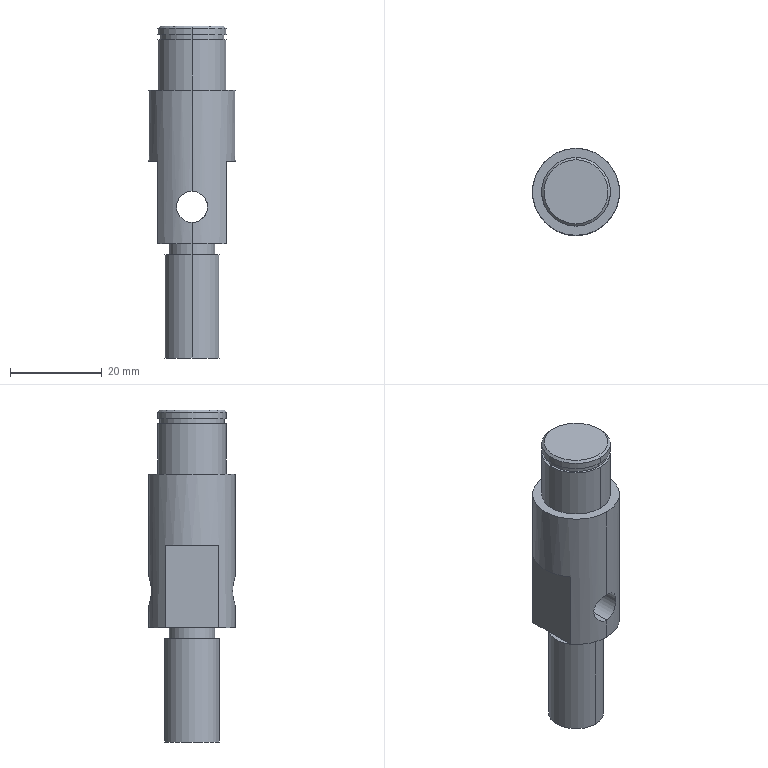Component | SolidWorks | DoubleFilmTransport-1_TensionConnectionAxis-1 | 1 solid | 27 faces | box 19 x 19 x 72.5 mm | volume 13431 mm3 | cylinder 14 | plane 11 | cone 2 | commonest cylinder face diameters 15 x4 6.8 x2 12 x2 10 x2 19 x2 14 x2
STEP:
#1=CARTESIAN_POINT('',(-15.145,10.074,3.252));
#2=VERTEX_POINT('',#1);
#3=CARTESIAN_POINT('',(-15.145,10.074,3.52));
#4=VERTEX_POINT('',#3);
#5=CARTESIAN_POINT('',(-15.145,10.074,3.252));
#6=CARTESIAN_POINT('',(-15.136,10.074,3.252));
#7=CARTESIAN_POINT('',(-15.127,10.074,3.253));
#8=CARTESIAN_POINT('',(-15.11,10.075,3.256));
#9=CARTESIAN_POINT('',(-15.101,10.076,3.259));
#10=CARTESIAN_POINT('',(-15.085,10.078,3.266));
#11=CARTESIAN_POINT('',(-15.077,10.08,3.27));
#12=CARTESIAN_POINT('',(-15.063,10.083,3.279));
#13=CARTESIAN_POINT('',(-15.056,10.084,3.285));
#14=CARTESIAN_POINT('',(-15.038,10.089,3.303));
#15=CARTESIAN_POINT('',(-15.028,10.092,3.318));
#16=CARTESIAN_POINT('',(-15.018,10.096,3.342));
#17=CARTESIAN_POINT('',(-15.015,10.097,3.351));
#18=CARTESIAN_POINT('',(-15.012,10.098,3.368));
#19=CARTESIAN_POINT('',(-15.011,10.099,3.377));
#20=CARTESIAN_POINT('',(-15.011,10.099,3.395));
#21=CARTESIAN_POINT('',(-15.012,10.098,3.404));
#22=CARTESIAN_POINT('',(-15.015,10.097,3.421));
#23=CARTESIAN_POINT('',(-15.018,10.096,3.429));
#24=CARTESIAN_POINT('',(-15.025,10.094,3.445));
#25=CARTESIAN_POINT('',(-15.029,10.092,3.453));
#26=CARTESIAN_POINT('',(-15.038,10.089,3.468));
#27=CARTESIAN_POINT('',(-15.044,10.088,3.474));
#28=CARTESIAN_POINT('',(-15.056,10.084,3.487));
#29=CARTESIAN_POINT('',(-15.063,10.083,3.492));
#30=CARTESIAN_POINT('',(-15.077,10.08,3.502));
#31=CARTESIAN_POINT('',(-15.085,10.078,3.506));
#32=CARTESIAN_POINT('',(-15.101,10.076,3.513));
#33=CARTESIAN_POINT('',(-15.11,10.075,3.515));
#34=CARTESIAN_POINT('',(-15.127,10.074,3.519));
#35=CARTESIAN_POINT('',(-15.136,10.074,3.52));
#36=CARTESIAN_POINT('',(-15.145,10.074,3.52));
#37=B_SPLINE_CURVE_WITH_KNOTS('',3,(#5,#6,#7,#8,#9,#10,#11,#12,#13,#14,#15,#16,#17,#18,#19,#20,#21,#22,#23,#24,#25,#26,#27,#28,#29,#30,#31,#32,#33,#34,#35,#36),.UNSPECIFIED.,.F.,.F.,(4,2,2,2,2,2,2,2,2,2,2,2,2,2,2,4),(0.,0.00067,0.00134,0.00201,0.00268,0.00402,0.00469,0.00536,0.00603,0.0067,0.00737,0.00804,0.00871,0.00938,0.01005,0.01072),.UNSPECIFIED.);
#38=EDGE_CURVE('',#2,#4,#37,.T.);
#39=ORIENTED_EDGE('',*,*,#38,.T.);
#40=CARTESIAN_POINT('',(-15.145,10.822,3.52));
#41=VERTEX_POINT('',#40);
#42=CARTESIAN_POINT('',(-15.145,10.822,3.52));
#43=DIRECTION('',(0.,1.,0.));
#44=VECTOR('',#43,39.37);
#45=LINE('',#42,#44);
#46=EDGE_CURVE('',#4,#41,#45,.T.);
#47=ORIENTED_EDGE('',*,*,#46,.T.);
#48=CARTESIAN_POINT('',(-15.145,10.822,3.252));
#49=VERTEX_POINT('',#48);
#50=CARTESIAN_POINT('',(-15.145,10.822,3.52));
#51=CARTESIAN_POINT('',(-15.136,10.822,3.52));
#52=CARTESIAN_POINT('',(-15.127,10.821,3.519));
#53=CARTESIAN_POINT('',(-15.11,10.82,3.515));
#54=CARTESIAN_POINT('',(-15.101,10.819,3.513));
#55=CARTESIAN_POINT('',(-15.085,10.817,3.506));
#56=CARTESIAN_POINT('',(-15.077,10.816,3.502));
#57=CARTESIAN_POINT('',(-15.063,10.813,3.492));
#58=CARTESIAN_POINT('',(-15.056,10.811,3.487));
#59=CARTESIAN_POINT('',(-15.044,10.808,3.474));
#60=CARTESIAN_POINT('',(-15.038,10.806,3.468));
#61=CARTESIAN_POINT('',(-15.029,10.803,3.453));
#62=CARTESIAN_POINT('',(-15.025,10.802,3.445));
#63=CARTESIAN_POINT('',(-15.018,10.8,3.429));
#64=CARTESIAN_POINT('',(-15.015,10.799,3.421));
#65=CARTESIAN_POINT('',(-15.012,10.797,3.404));
#66=CARTESIAN_POINT('',(-15.011,10.797,3.395));
#67=CARTESIAN_POINT('',(-15.011,10.797,3.377));
#68=CARTESIAN_POINT('',(-15.012,10.797,3.368));
#69=CARTESIAN_POINT('',(-15.015,10.799,3.351));
#70=CARTESIAN_POINT('',(-15.018,10.8,3.342));
#71=CARTESIAN_POINT('',(-15.025,10.802,3.326));
#72=CARTESIAN_POINT('',(-15.029,10.803,3.319));
#73=CARTESIAN_POINT('',(-15.038,10.806,3.304));
#74=CARTESIAN_POINT('',(-15.044,10.808,3.297));
#75=CARTESIAN_POINT('',(-15.056,10.811,3.285));
#76=CARTESIAN_POINT('',(-15.063,10.813,3.279));
#77=CARTESIAN_POINT('',(-15.078,10.816,3.27));
#78=CARTESIAN_POINT('',(-15.085,10.817,3.266));
#79=CARTESIAN_POINT('',(-15.101,10.819,3.259));
#80=CARTESIAN_POINT('',(-15.11,10.82,3.256));
#81=CARTESIAN_POINT('',(-15.127,10.821,3.253));
#82=CARTESIAN_POINT('',(-15.136,10.822,3.252));
#83=CARTESIAN_POINT('',(-15.145,10.822,3.252));
#84=B_SPLINE_CURVE_WITH_KNOTS('',3,(#50,#51,#52,#53,#54,#55,#56,#57,#58,#59,#60,#61,#62,#63,#64,#65,#66,#67,#68,#69,#70,#71,#72,#73,#74,#75,#76,#77,#78,#79,#80,#81,#82,#83),.UNSPECIFIED.,.F.,.F.,(4,2,2,2,2,2,2,2,2,2,2,2,2,2,2,2,4),(0.01072,0.01139,0.01206,0.01273,0.0134,0.01407,0.01474,0.01541,0.01608,0.01675,0.01742,0.01809,0.01876,0.01943,0.0201,0.02077,0.02144),.UNSPECIFIED.);
#85=EDGE_CURVE('',#41,#49,#84,.T.);
#86=ORIENTED_EDGE('',*,*,#85,.T.);
#87=CARTESIAN_POINT('',(-15.145,10.822,3.252));
#88=DIRECTION('',(0.,1.,0.));
#89=VECTOR('',#88,39.37);
#90=LINE('',#87,#89);
#91=EDGE_CURVE('',#2,#49,#90,.T.);
#92=ORIENTED_EDGE('',*,*,#91,.F.);
#93=EDGE_LOOP('',(#39,#47,#86,#92));
#94=FACE_OUTER_BOUND('',#93,.T.);
#95=CARTESIAN_POINT('',(-15.145,10.822,3.386));
#96=DIRECTION('',(0.,1.,0.));
#97=DIRECTION('',(0.,0.,-1.));
#98=AXIS2_PLACEMENT_3D('',#95,#96,#97);
#99=CYLINDRICAL_SURFACE('',#98,0.1339);
#100=ADVANCED_FACE('',(#94),#99,.F.);
#101=CARTESIAN_POINT('',(-15.145,10.684,2.087));
#102=VERTEX_POINT('',#101);
#103=CARTESIAN_POINT('',(-15.145,10.212,2.087));
#104=VERTEX_POINT('',#103);
#105=CARTESIAN_POINT('',(-15.145,10.448,2.087));
#106=DIRECTION('',(0.,0.,1.));
#107=DIRECTION('',(0.,-1.,0.));
#108=AXIS2_PLACEMENT_3D('',#105,#106,#107);
#109=CIRCLE('',#108,0.2362);
#110=EDGE_CURVE('',#102,#104,#109,.T.);
#111=ORIENTED_EDGE('',*,*,#110,.T.);
#112=CARTESIAN_POINT('',(-15.145,10.212,2.972));
#113=VERTEX_POINT('',#112);
#114=CARTESIAN_POINT('',(-15.145,10.212,2.087));
#115=DIRECTION('',(0.,0.,1.));
#116=VECTOR('',#115,39.37);
#117=LINE('',#114,#116);
#118=EDGE_CURVE('',#104,#113,#117,.T.);
#119=ORIENTED_EDGE('',*,*,#118,.T.);
#120=CARTESIAN_POINT('',(-15.145,10.684,2.972));
#121=VERTEX_POINT('',#120);
#122=CARTESIAN_POINT('',(-15.145,10.448,2.972));
#123=DIRECTION('',(0.,0.,1.));
#124=DIRECTION('',(0.,-1.,0.));
#125=AXIS2_PLACEMENT_3D('',#122,#123,#124);
#126=CIRCLE('',#125,0.2362);
#127=EDGE_CURVE('',#121,#113,#126,.T.);
#128=ORIENTED_EDGE('',*,*,#127,.F.);
#129=CARTESIAN_POINT('',(-15.145,10.684,2.087));
#130=DIRECTION('',(0.,0.,1.));
#131=VECTOR('',#130,39.37);
#132=LINE('',#129,#131);
#133=EDGE_CURVE('',#102,#121,#132,.T.);
#134=ORIENTED_EDGE('',*,*,#133,.F.);
#135=EDGE_LOOP('',(#111,#119,#128,#134));
#136=FACE_OUTER_BOUND('',#135,.T.);
#137=CARTESIAN_POINT('',(-15.145,10.448,2.087));
#138=DIRECTION('',(0.,0.,1.));
#139=DIRECTION('',(0.,1.,0.));
#140=AXIS2_PLACEMENT_3D('',#137,#138,#139);
#141=CYLINDRICAL_SURFACE('',#140,0.2362);
#142=ADVANCED_FACE('',(#136),#141,.T.);
#143=CARTESIAN_POINT('',(-15.145,10.251,2.972));
#144=VERTEX_POINT('',#143);
#145=CARTESIAN_POINT('',(-15.145,10.645,2.972));
#146=VERTEX_POINT('',#145);
#147=CARTESIAN_POINT('',(-15.145,10.448,2.972));
#148=DIRECTION('',(0.,0.,-1.));
#149=DIRECTION('',(0.,-1.,0.));
#150=AXIS2_PLACEMENT_3D('',#147,#148,#149);
#151=CIRCLE('',#150,0.1969);
#152=EDGE_CURVE('',#144,#146,#151,.T.);
#153=ORIENTED_EDGE('',*,*,#152,.F.);
#154=CARTESIAN_POINT('',(-15.145,10.251,3.071));
#155=VERTEX_POINT('',#154);
#156=CARTESIAN_POINT('',(-15.145,10.251,2.972));
#157=DIRECTION('',(0.,0.,1.));
#158=VECTOR('',#157,39.37);
#159=LINE('',#156,#158);
#160=EDGE_CURVE('',#144,#155,#159,.T.);
#161=ORIENTED_EDGE('',*,*,#160,.T.);
#162=CARTESIAN_POINT('',(-15.145,10.645,3.071));
#163=VERTEX_POINT('',#162);
#164=CARTESIAN_POINT('',(-15.145,10.448,3.071));
#165=DIRECTION('',(0.,0.,-1.));
#166=DIRECTION('',(0.,-1.,0.));
#167=AXIS2_PLACEMENT_3D('',#164,#165,#166);
#168=CIRCLE('',#167,0.1969);
#169=EDGE_CURVE('',#155,#163,#168,.T.);
#170=ORIENTED_EDGE('',*,*,#169,.T.);
#171=CARTESIAN_POINT('',(-15.145,10.645,2.972));
#172=DIRECTION('',(0.,0.,1.));
#173=VECTOR('',#172,39.37);
#174=LINE('',#171,#173);
#175=EDGE_CURVE('',#146,#163,#174,.T.);
#176=ORIENTED_EDGE('',*,*,#175,.F.);
#177=EDGE_LOOP('',(#153,#161,#170,#176));
#178=FACE_OUTER_BOUND('',#177,.T.);
#179=CARTESIAN_POINT('',(-15.145,10.448,2.972));
#180=DIRECTION('',(0.,0.,1.));
#181=DIRECTION('',(0.,1.,0.));
#182=AXIS2_PLACEMENT_3D('',#179,#180,#181);
#183=CYLINDRICAL_SURFACE('',#182,0.1969);
#184=ADVANCED_FACE('',(#178),#183,.T.);
#185=CARTESIAN_POINT('',(-15.44,10.218,3.071));
#186=VERTEX_POINT('',#185);
#187=CARTESIAN_POINT('',(-15.145,10.074,3.071));
#188=VERTEX_POINT('',#187);
#189=CARTESIAN_POINT('',(-15.145,10.448,3.071));
#190=DIRECTION('',(0.,0.,1.));
#191=DIRECTION('',(0.,-1.,0.));
#192=AXIS2_PLACEMENT_3D('',#189,#190,#191);
#193=CIRCLE('',#192,0.374);
#194=EDGE_CURVE('',#186,#188,#193,.T.);
#195=ORIENTED_EDGE('',*,*,#194,.T.);
#196=CARTESIAN_POINT('',(-15.145,10.074,3.071));
#197=DIRECTION('',(0.,0.,1.));
#198=VECTOR('',#197,39.37);
#199=LINE('',#196,#198);
#200=EDGE_CURVE('',#188,#2,#199,.T.);
#201=ORIENTED_EDGE('',*,*,#200,.T.);
#202=CARTESIAN_POINT('',(-15.145,10.074,3.52));
#203=CARTESIAN_POINT('',(-15.154,10.074,3.52));
#204=CARTESIAN_POINT('',(-15.162,10.074,3.519));
#205=CARTESIAN_POINT('',(-15.18,10.075,3.515));
#206=CARTESIAN_POINT('',(-15.188,10.076,3.513));
#207=CARTESIAN_POINT('',(-15.204,10.078,3.506));
#208=CARTESIAN_POINT('',(-15.212,10.08,3.502));
#209=CARTESIAN_POINT('',(-15.227,10.083,3.492));
#210=CARTESIAN_POINT('',(-15.233,10.084,3.487));
#211=CARTESIAN_POINT('',(-15.246,10.088,3.474));
#212=CARTESIAN_POINT('',(-15.251,10.089,3.468));
#213=CARTESIAN_POINT('',(-15.261,10.092,3.453));
#214=CARTESIAN_POINT('',(-15.265,10.094,3.445));
#215=CARTESIAN_POINT('',(-15.272,10.096,3.429));
#216=CARTESIAN_POINT('',(-15.274,10.097,3.421));
#217=CARTESIAN_POINT('',(-15.278,10.098,3.404));
#218=CARTESIAN_POINT('',(-15.279,10.099,3.395));
#219=CARTESIAN_POINT('',(-15.279,10.099,3.377));
#220=CARTESIAN_POINT('',(-15.278,10.098,3.368));
#221=CARTESIAN_POINT('',(-15.274,10.097,3.351));
#222=CARTESIAN_POINT('',(-15.272,10.096,3.342));
#223=CARTESIAN_POINT('',(-15.265,10.094,3.326));
#224=CARTESIAN_POINT('',(-15.261,10.092,3.319));
#225=CARTESIAN_POINT('',(-15.251,10.089,3.304));
#226=CARTESIAN_POINT('',(-15.246,10.088,3.297));
#227=CARTESIAN_POINT('',(-15.233,10.084,3.285));
#228=CARTESIAN_POINT('',(-15.226,10.083,3.279));
#229=CARTESIAN_POINT('',(-15.212,10.08,3.27));
#230=CARTESIAN_POINT('',(-15.204,10.078,3.266));
#231=CARTESIAN_POINT('',(-15.188,10.076,3.259));
#232=CARTESIAN_POINT('',(-15.18,10.075,3.256));
#233=CARTESIAN_POINT('',(-15.162,10.074,3.253));
#234=CARTESIAN_POINT('',(-15.154,10.074,3.252));
#235=CARTESIAN_POINT('',(-15.145,10.074,3.252));
#236=B_SPLINE_CURVE_WITH_KNOTS('',3,(#202,#203,#204,#205,#206,#207,#208,#209,#210,#211,#212,#213,#214,#215,#216,#217,#218,#219,#220,#221,#222,#223,#224,#225,#226,#227,#228,#229,#230,#231,#232,#233,#234,#235),.UNSPECIFIED.,.F.,.F.,(4,2,2,2,2,2,2,2,2,2,2,2,2,2,2,2,4),(0.01072,0.01139,0.01206,0.01273,0.0134,0.01407,0.01474,0.01541,0.01608,0.01675,0.01742,0.01809,0.01876,0.01943,0.0201,0.02077,0.02144),.UNSPECIFIED.);
#237=EDGE_CURVE('',#4,#2,#236,.T.);
#238=ORIENTED_EDGE('',*,*,#237,.F.);
#239=CARTESIAN_POINT('',(-15.145,10.074,4.39));
#240=VERTEX_POINT('',#239);
#241=CARTESIAN_POINT('',(-15.145,10.074,3.071));
#242=DIRECTION('',(0.,0.,1.));
#243=VECTOR('',#242,39.37);
#244=LINE('',#241,#243);
#245=EDGE_CURVE('',#4,#240,#244,.T.);
#246=ORIENTED_EDGE('',*,*,#245,.T.);
#247=CARTESIAN_POINT('',(-15.145,10.822,4.39));
#248=VERTEX_POINT('',#247);
#249=CARTESIAN_POINT('',(-15.145,10.448,4.39));
#250=DIRECTION('',(0.,0.,1.));
#251=DIRECTION('',(0.,-1.,0.));
#252=AXIS2_PLACEMENT_3D('',#249,#250,#251);
#253=CIRCLE('',#252,0.374);
#254=EDGE_CURVE('',#248,#240,#253,.T.);
#255=ORIENTED_EDGE('',*,*,#254,.F.);
#256=CARTESIAN_POINT('',(-15.145,10.822,3.071));
#257=DIRECTION('',(0.,0.,1.));
#258=VECTOR('',#257,39.37);
#259=LINE('',#256,#258);
#260=EDGE_CURVE('',#41,#248,#259,.T.);
#261=ORIENTED_EDGE('',*,*,#260,.F.);
#262=CARTESIAN_POINT('',(-15.145,10.822,3.252));
#263=CARTESIAN_POINT('',(-15.154,10.822,3.252));
#264=CARTESIAN_POINT('',(-15.162,10.821,3.253));
#265=CARTESIAN_POINT('',(-15.18,10.82,3.256));
#266=CARTESIAN_POINT('',(-15.188,10.819,3.259));
#267=CARTESIAN_POINT('',(-15.204,10.817,3.266));
#268=CARTESIAN_POINT('',(-15.212,10.816,3.27));
#269=CARTESIAN_POINT('',(-15.227,10.813,3.279));
#270=CARTESIAN_POINT('',(-15.233,10.811,3.285));
#271=CARTESIAN_POINT('',(-15.252,10.806,3.303));
#272=CARTESIAN_POINT('',(-15.262,10.803,3.318));
#273=CARTESIAN_POINT('',(-15.272,10.8,3.342));
#274=CARTESIAN_POINT('',(-15.274,10.799,3.351));
#275=CARTESIAN_POINT('',(-15.278,10.797,3.368));
#276=CARTESIAN_POINT('',(-15.279,10.797,3.377));
#277=CARTESIAN_POINT('',(-15.279,10.797,3.395));
#278=CARTESIAN_POINT('',(-15.278,10.797,3.404));
#279=CARTESIAN_POINT('',(-15.274,10.799,3.421));
#280=CARTESIAN_POINT('',(-15.272,10.8,3.429));
#281=CARTESIAN_POINT('',(-15.265,10.802,3.445));
#282=CARTESIAN_POINT('',(-15.261,10.803,3.453));
#283=CARTESIAN_POINT('',(-15.251,10.806,3.468));
#284=CARTESIAN_POINT('',(-15.246,10.808,3.474));
#285=CARTESIAN_POINT('',(-15.233,10.811,3.487));
#286=CARTESIAN_POINT('',(-15.227,10.813,3.492));
#287=CARTESIAN_POINT('',(-15.212,10.816,3.502));
#288=CARTESIAN_POINT('',(-15.204,10.817,3.506));
#289=CARTESIAN_POINT('',(-15.188,10.819,3.513));
#290=CARTESIAN_POINT('',(-15.18,10.82,3.515));
#291=CARTESIAN_POINT('',(-15.162,10.821,3.519));
#292=CARTESIAN_POINT('',(-15.154,10.822,3.52));
#293=CARTESIAN_POINT('',(-15.145,10.822,3.52));
#294=B_SPLINE_CURVE_WITH_KNOTS('',3,(#262,#263,#264,#265,#266,#267,#268,#269,#270,#271,#272,#273,#274,#275,#276,#277,#278,#279,#280,#281,#282,#283,#284,#285,#286,#287,#288,#289,#290,#291,#292,#293),.UNSPECIFIED.,.F.,.F.,(4,2,2,2,2,2,2,2,2,2,2,2,2,2,2,4),(0.,0.00067,0.00134,0.00201,0.00268,0.00402,0.00469,0.00536,0.00603,0.0067,0.00737,0.00804,0.00871,0.00938,0.01005,0.01072),.UNSPECIFIED.);
#295=EDGE_CURVE('',#49,#41,#294,.T.);
#296=ORIENTED_EDGE('',*,*,#295,.F.);
#297=CARTESIAN_POINT('',(-15.145,10.822,3.071));
#298=VERTEX_POINT('',#297);
#299=CARTESIAN_POINT('',(-15.145,10.822,3.071));
#300=DIRECTION('',(0.,0.,1.));
#301=VECTOR('',#300,39.37);
#302=LINE('',#299,#301);
#303=EDGE_CURVE('',#298,#49,#302,.T.);
#304=ORIENTED_EDGE('',*,*,#303,.F.);
#305=CARTESIAN_POINT('',(-15.44,10.677,3.071));
#306=VERTEX_POINT('',#305);
#307=CARTESIAN_POINT('',(-15.145,10.448,3.071));
#308=DIRECTION('',(0.,0.,1.));
#309=DIRECTION('',(0.,-1.,0.));
#310=AXIS2_PLACEMENT_3D('',#307,#308,#309);
#311=CIRCLE('',#310,0.374);
#312=EDGE_CURVE('',#298,#306,#311,.T.);
#313=ORIENTED_EDGE('',*,*,#312,.T.);
#314=CARTESIAN_POINT('',(-15.44,10.677,3.78));
#315=VERTEX_POINT('',#314);
#316=CARTESIAN_POINT('',(-15.44,10.677,3.78));
#317=DIRECTION('',(0.,0.,-1.));
#318=VECTOR('',#317,39.37);
#319=LINE('',#316,#318);
#320=EDGE_CURVE('',#315,#306,#319,.T.);
#321=ORIENTED_EDGE('',*,*,#320,.F.);
#322=CARTESIAN_POINT('',(-15.44,10.218,3.78));
#323=VERTEX_POINT('',#322);
#324=CARTESIAN_POINT('',(-15.145,10.448,3.78));
#325=DIRECTION('',(0.,0.,-1.));
#326=DIRECTION('',(0.,-1.,0.));
#327=AXIS2_PLACEMENT_3D('',#324,#325,#326);
#328=CIRCLE('',#327,0.374);
#329=EDGE_CURVE('',#323,#315,#328,.T.);
#330=ORIENTED_EDGE('',*,*,#329,.F.);
#331=CARTESIAN_POINT('',(-15.44,10.218,3.78));
#332=DIRECTION('',(0.,0.,-1.));
#333=VECTOR('',#332,39.37);
#334=LINE('',#331,#333);
#335=EDGE_CURVE('',#323,#186,#334,.T.);
#336=ORIENTED_EDGE('',*,*,#335,.T.);
#337=EDGE_LOOP('',(#195,#201,#238,#246,#255,#261,#296,#304,#313,#321,#330,#336));
#338=FACE_OUTER_BOUND('',#337,.T.);
#339=CARTESIAN_POINT('',(-15.145,10.448,3.071));
#340=DIRECTION('',(0.,0.,1.));
#341=DIRECTION('',(0.,1.,0.));
#342=AXIS2_PLACEMENT_3D('',#339,#340,#341);
#343=CYLINDRICAL_SURFACE('',#342,0.374);
#344=ADVANCED_FACE('',(#338),#343,.T.);
#345=CARTESIAN_POINT('',(-15.145,10.743,4.39));
#346=VERTEX_POINT('',#345);
#347=CARTESIAN_POINT('',(-15.145,10.152,4.39));
#348=VERTEX_POINT('',#347);
#349=CARTESIAN_POINT('',(-15.145,10.448,4.39));
#350=DIRECTION('',(0.,0.,1.));
#351=DIRECTION('',(0.,-1.,0.));
#352=AXIS2_PLACEMENT_3D('',#349,#350,#351);
#353=CIRCLE('',#352,0.2953);
#354=EDGE_CURVE('',#346,#348,#353,.T.);
#355=ORIENTED_EDGE('',*,*,#354,.T.);
#356=CARTESIAN_POINT('',(-15.145,10.152,4.823));
#357=VERTEX_POINT('',#356);
#358=CARTESIAN_POINT('',(-15.145,10.152,4.39));
#359=DIRECTION('',(0.,0.,1.));
#360=VECTOR('',#359,39.37);
#361=LINE('',#358,#360);
#362=EDGE_CURVE('',#348,#357,#361,.T.);
#363=ORIENTED_EDGE('',*,*,#362,.T.);
#364=CARTESIAN_POINT('',(-15.145,10.743,4.823));
#365=VERTEX_POINT('',#364);
#366=CARTESIAN_POINT('',(-15.145,10.448,4.823));
#367=DIRECTION('',(0.,0.,1.));
#368=DIRECTION('',(0.,-1.,0.));
#369=AXIS2_PLACEMENT_3D('',#366,#367,#368);
#370=CIRCLE('',#369,0.2953);
#371=EDGE_CURVE('',#365,#357,#370,.T.);
#372=ORIENTED_EDGE('',*,*,#371,.F.);
#373=CARTESIAN_POINT('',(-15.145,10.743,4.39));
#374=DIRECTION('',(0.,0.,1.));
#375=VECTOR('',#374,39.37);
#376=LINE('',#373,#375);
#377=EDGE_CURVE('',#346,#365,#376,.T.);
#378=ORIENTED_EDGE('',*,*,#377,.F.);
#379=EDGE_LOOP('',(#355,#363,#372,#378));
#380=FACE_OUTER_BOUND('',#379,.T.);
#381=CARTESIAN_POINT('',(-15.145,10.448,4.39));
#382=DIRECTION('',(0.,0.,1.));
#383=DIRECTION('',(0.,1.,0.));
#384=AXIS2_PLACEMENT_3D('',#381,#382,#383);
#385=CYLINDRICAL_SURFACE('',#384,0.2953);
#386=ADVANCED_FACE('',(#380),#385,.T.);
#387=CARTESIAN_POINT('',(-15.145,10.172,4.823));
#388=VERTEX_POINT('',#387);
#389=CARTESIAN_POINT('',(-15.145,10.723,4.823));
#390=VERTEX_POINT('',#389);
#391=CARTESIAN_POINT('',(-15.145,10.448,4.823));
#392=DIRECTION('',(0.,0.,-1.));
#393=DIRECTION('',(0.,-1.,0.));
#394=AXIS2_PLACEMENT_3D('',#391,#392,#393);
#395=CIRCLE('',#394,0.2756);
#396=EDGE_CURVE('',#388,#390,#395,.T.);
#397=ORIENTED_EDGE('',*,*,#396,.F.);
#398=CARTESIAN_POINT('',(-15.145,10.172,4.866));
#399=VERTEX_POINT('',#398);
#400=CARTESIAN_POINT('',(-15.145,10.172,4.823));
#401=DIRECTION('',(0.,0.,1.));
#402=VECTOR('',#401,39.37);
#403=LINE('',#400,#402);
#404=EDGE_CURVE('',#388,#399,#403,.T.);
#405=ORIENTED_EDGE('',*,*,#404,.T.);
#406=CARTESIAN_POINT('',(-15.145,10.723,4.866));
#407=VERTEX_POINT('',#406);
#408=CARTESIAN_POINT('',(-15.145,10.448,4.866));
#409=DIRECTION('',(0.,0.,-1.));
#410=DIRECTION('',(0.,-1.,0.));
#411=AXIS2_PLACEMENT_3D('',#408,#409,#410);
#412=CIRCLE('',#411,0.2756);
#413=EDGE_CURVE('',#399,#407,#412,.T.);
#414=ORIENTED_EDGE('',*,*,#413,.T.);
#415=CARTESIAN_POINT('',(-15.145,10.723,4.823));
#416=DIRECTION('',(0.,0.,1.));
#417=VECTOR('',#416,39.37);
#418=LINE('',#415,#417);
#419=EDGE_CURVE('',#390,#407,#418,.T.);
#420=ORIENTED_EDGE('',*,*,#419,.F.);
#421=EDGE_LOOP('',(#397,#405,#414,#420));
#422=FACE_OUTER_BOUND('',#421,.T.);
#423=CARTESIAN_POINT('',(-15.145,10.448,4.823));
#424=DIRECTION('',(0.,0.,1.));
#425=DIRECTION('',(0.,1.,0.));
#426=AXIS2_PLACEMENT_3D('',#423,#424,#425);
#427=CYLINDRICAL_SURFACE('',#426,0.2756);
#428=ADVANCED_FACE('',(#422),#427,.T.);
#429=CARTESIAN_POINT('',(-15.145,10.152,4.866));
#430=VERTEX_POINT('',#429);
#431=CARTESIAN_POINT('',(-15.145,10.743,4.866));
#432=VERTEX_POINT('',#431);
#433=CARTESIAN_POINT('',(-15.145,10.448,4.866));
#434=DIRECTION('',(0.,0.,-1.));
#435=DIRECTION('',(0.,-1.,0.));
#436=AXIS2_PLACEMENT_3D('',#433,#434,#435);
#437=CIRCLE('',#436,0.2953);
#438=EDGE_CURVE('',#430,#432,#437,.T.);
#439=ORIENTED_EDGE('',*,*,#438,.F.);
#440=CARTESIAN_POINT('',(-15.145,10.152,4.921));
#441=VERTEX_POINT('',#440);
#442=CARTESIAN_POINT('',(-15.145,10.152,4.866));
#443=DIRECTION('',(0.,0.,1.));
#444=VECTOR('',#443,39.37);
#445=LINE('',#442,#444);
#446=EDGE_CURVE('',#430,#441,#445,.T.);
#447=ORIENTED_EDGE('',*,*,#446,.T.);
#448=CARTESIAN_POINT('',(-15.145,10.743,4.921));
#449=VERTEX_POINT('',#448);
#450=CARTESIAN_POINT('',(-15.145,10.448,4.921));
#451=DIRECTION('',(0.,0.,-1.));
#452=DIRECTION('',(0.,-1.,0.));
#453=AXIS2_PLACEMENT_3D('',#450,#451,#452);
#454=CIRCLE('',#453,0.2953);
#455=EDGE_CURVE('',#441,#449,#454,.T.);
#456=ORIENTED_EDGE('',*,*,#455,.T.);
#457=CARTESIAN_POINT('',(-15.145,10.743,4.866));
#458=DIRECTION('',(0.,0.,1.));
#459=VECTOR('',#458,39.37);
#460=LINE('',#457,#459);
#461=EDGE_CURVE('',#432,#449,#460,.T.);
#462=ORIENTED_EDGE('',*,*,#461,.F.);
#463=EDGE_LOOP('',(#439,#447,#456,#462));
#464=FACE_OUTER_BOUND('',#463,.T.);
#465=CARTESIAN_POINT('',(-15.145,10.448,4.866));
#466=DIRECTION('',(0.,0.,1.));
#467=DIRECTION('',(0.,1.,0.));
#468=AXIS2_PLACEMENT_3D('',#465,#466,#467);
#469=CYLINDRICAL_SURFACE('',#468,0.2953);
#470=ADVANCED_FACE('',(#464),#469,.T.);
#471=CARTESIAN_POINT('',(-15.145,10.172,4.941));
#472=VERTEX_POINT('',#471);
#473=CARTESIAN_POINT('',(-15.145,10.723,4.941));
#474=VERTEX_POINT('',#473);
#475=CARTESIAN_POINT('',(-15.145,10.448,4.941));
#476=DIRECTION('',(0.,0.,-1.));
#477=DIRECTION('',(0.,-1.,0.));
#478=AXIS2_PLACEMENT_3D('',#475,#476,#477);
#479=CIRCLE('',#478,0.2756);
#480=EDGE_CURVE('',#472,#474,#479,.T.);
#481=ORIENTED_EDGE('',*,*,#480,.T.);
#482=CARTESIAN_POINT('',(-15.145,10.743,4.921));
#483=DIRECTION('',(-0.,0.7071,-0.7071));
#484=VECTOR('',#483,39.37);
#485=LINE('',#482,#484);
#486=EDGE_CURVE('',#474,#449,#485,.T.);
#487=ORIENTED_EDGE('',*,*,#486,.T.);
#488=ORIENTED_EDGE('',*,*,#455,.F.);
#489=CARTESIAN_POINT('',(-15.145,10.152,4.921));
#490=DIRECTION('',(-0.,-0.7071,-0.7071));
#491=VECTOR('',#490,39.37);
#492=LINE('',#489,#491);
#493=EDGE_CURVE('',#472,#441,#492,.T.);
#494=ORIENTED_EDGE('',*,*,#493,.F.);
#495=EDGE_LOOP('',(#481,#487,#488,#494));
#496=FACE_OUTER_BOUND('',#495,.T.);
#497=CARTESIAN_POINT('',(-15.145,10.448,4.921));
#498=DIRECTION('',(0.,0.,-1.));
#499=DIRECTION('',(0.,-1.,0.));
#500=AXIS2_PLACEMENT_3D('',#497,#498,#499);
#501=CONICAL_SURFACE('',#500,0.2953,0.7854);
#502=ADVANCED_FACE('',(#496),#501,.T.);
#503=ORIENTED_EDGE('',*,*,#486,.F.);
#504=CARTESIAN_POINT('',(-15.145,10.448,4.941));
#505=DIRECTION('',(0.,0.,-1.));
#506=DIRECTION('',(0.,-1.,0.));
#507=AXIS2_PLACEMENT_3D('',#504,#505,#506);
#508=CIRCLE('',#507,0.2756);
#509=EDGE_CURVE('',#474,#472,#508,.T.);
#510=ORIENTED_EDGE('',*,*,#509,.T.);
#511=ORIENTED_EDGE('',*,*,#493,.T.);
#512=CARTESIAN_POINT('',(-15.145,10.448,4.921));
#513=DIRECTION('',(0.,0.,-1.));
#514=DIRECTION('',(0.,-1.,0.));
#515=AXIS2_PLACEMENT_3D('',#512,#513,#514);
#516=CIRCLE('',#515,0.2953);
#517=EDGE_CURVE('',#449,#441,#516,.T.);
#518=ORIENTED_EDGE('',*,*,#517,.F.);
#519=EDGE_LOOP('',(#503,#510,#511,#518));
#520=FACE_OUTER_BOUND('',#519,.T.);
#521=CARTESIAN_POINT('',(-15.145,10.448,4.921));
#522=DIRECTION('',(0.,0.,-1.));
#523=DIRECTION('',(0.,-1.,0.));
#524=AXIS2_PLACEMENT_3D('',#521,#522,#523);
#525=CONICAL_SURFACE('',#524,0.2953,0.7854);
#526=ADVANCED_FACE('',(#520),#525,.T.);
#527=ORIENTED_EDGE('',*,*,#480,.F.);
#528=ORIENTED_EDGE('',*,*,#509,.F.);
#529=EDGE_LOOP('',(#527,#528));
#530=FACE_OUTER_BOUND('',#529,.T.);
#531=CARTESIAN_POINT('',(-15.145,10.448,4.941));
#532=DIRECTION('',(0.,0.,-1.));
#533=DIRECTION('',(-0.,-1.,0.));
#534=AXIS2_PLACEMENT_3D('',#531,#532,#533);
#535=PLANE('',#534);
#536=ADVANCED_FACE('',(#530),#535,.F.);
#537=ORIENTED_EDGE('',*,*,#446,.F.);
#538=CARTESIAN_POINT('',(-15.145,10.448,4.866));
#539=DIRECTION('',(0.,0.,-1.));
#540=DIRECTION('',(0.,-1.,0.));
#541=AXIS2_PLACEMENT_3D('',#538,#539,#540);
#542=CIRCLE('',#541,0.2953);
#543=EDGE_CURVE('',#432,#430,#542,.T.);
#544=ORIENTED_EDGE('',*,*,#543,.F.);
#545=ORIENTED_EDGE('',*,*,#461,.T.);
#546=ORIENTED_EDGE('',*,*,#517,.T.);
#547=EDGE_LOOP('',(#537,#544,#545,#546));
#548=FACE_OUTER_BOUND('',#547,.T.);
#549=CARTESIAN_POINT('',(-15.145,10.448,4.866));
#550=DIRECTION('',(0.,0.,1.));
#551=DIRECTION('',(0.,1.,0.));
#552=AXIS2_PLACEMENT_3D('',#549,#550,#551);
#553=CYLINDRICAL_SURFACE('',#552,0.2953);
#554=ADVANCED_FACE('',(#548),#553,.T.);
#555=CARTESIAN_POINT('',(-15.145,10.448,4.866));
#556=DIRECTION('',(0.,0.,-1.));
#557=DIRECTION('',(0.,-1.,0.));
#558=AXIS2_PLACEMENT_3D('',#555,#556,#557);
#559=CIRCLE('',#558,0.2756);
#560=EDGE_CURVE('',#407,#399,#559,.T.);
#561=ORIENTED_EDGE('',*,*,#560,.F.);
#562=ORIENTED_EDGE('',*,*,#413,.F.);
#563=EDGE_LOOP('',(#561,#562));
#564=FACE_BOUND('',#563,.T.);
#565=ORIENTED_EDGE('',*,*,#543,.T.);
#566=ORIENTED_EDGE('',*,*,#438,.T.);
#567=EDGE_LOOP('',(#565,#566));
#568=FACE_OUTER_BOUND('',#567,.T.);
#569=CARTESIAN_POINT('',(-15.145,10.448,4.866));
#570=DIRECTION('',(0.,0.,-1.));
#571=DIRECTION('',(-0.,-1.,0.));
#572=AXIS2_PLACEMENT_3D('',#569,#570,#571);
#573=PLANE('',#572);
#574=ADVANCED_FACE('',(#564,#568),#573,.T.);
#575=ORIENTED_EDGE('',*,*,#404,.F.);
#576=CARTESIAN_POINT('',(-15.145,10.448,4.823));
#577=DIRECTION('',(0.,0.,-1.));
#578=DIRECTION('',(0.,-1.,0.));
#579=AXIS2_PLACEMENT_3D('',#576,#577,#578);
#580=CIRCLE('',#579,0.2756);
#581=EDGE_CURVE('',#390,#388,#580,.T.);
#582=ORIENTED_EDGE('',*,*,#581,.F.);
#583=ORIENTED_EDGE('',*,*,#419,.T.);
#584=ORIENTED_EDGE('',*,*,#560,.T.);
#585=EDGE_LOOP('',(#575,#582,#583,#584));
#586=FACE_OUTER_BOUND('',#585,.T.);
#587=CARTESIAN_POINT('',(-15.145,10.448,4.823));
#588=DIRECTION('',(0.,0.,1.));
#589=DIRECTION('',(0.,1.,0.));
#590=AXIS2_PLACEMENT_3D('',#587,#588,#589);
#591=CYLINDRICAL_SURFACE('',#590,0.2756);
#592=ADVANCED_FACE('',(#586),#591,.T.);
#593=ORIENTED_EDGE('',*,*,#362,.F.);
#594=CARTESIAN_POINT('',(-15.145,10.448,4.39));
#595=DIRECTION('',(0.,0.,1.));
#596=DIRECTION('',(0.,-1.,0.));
#597=AXIS2_PLACEMENT_3D('',#594,#595,#596);
#598=CIRCLE('',#597,0.2953);
#599=EDGE_CURVE('',#348,#346,#598,.T.);
#600=ORIENTED_EDGE('',*,*,#599,.T.);
#601=ORIENTED_EDGE('',*,*,#377,.T.);
#602=CARTESIAN_POINT('',(-15.145,10.448,4.823));
#603=DIRECTION('',(0.,0.,1.));
#604=DIRECTION('',(0.,-1.,0.));
#605=AXIS2_PLACEMENT_3D('',#602,#603,#604);
#606=CIRCLE('',#605,0.2953);
#607=EDGE_CURVE('',#357,#365,#606,.T.);
#608=ORIENTED_EDGE('',*,*,#607,.F.);
#609=EDGE_LOOP('',(#593,#600,#601,#608));
#610=FACE_OUTER_BOUND('',#609,.T.);
#611=CARTESIAN_POINT('',(-15.145,10.448,4.39));
#612=DIRECTION('',(0.,0.,1.));
#613=DIRECTION('',(0.,1.,0.));
#614=AXIS2_PLACEMENT_3D('',#611,#612,#613);
#615=CYLINDRICAL_SURFACE('',#614,0.2953);
#616=ADVANCED_FACE('',(#610),#615,.T.);
#617=ORIENTED_EDGE('',*,*,#581,.T.);
#618=ORIENTED_EDGE('',*,*,#396,.T.);
#619=EDGE_LOOP('',(#617,#618));
#620=FACE_BOUND('',#619,.T.);
#621=ORIENTED_EDGE('',*,*,#371,.T.);
#622=ORIENTED_EDGE('',*,*,#607,.T.);
#623=EDGE_LOOP('',(#621,#622));
#624=FACE_OUTER_BOUND('',#623,.T.);
#625=CARTESIAN_POINT('',(-15.145,10.448,4.823));
#626=DIRECTION('',(0.,0.,-1.));
#627=DIRECTION('',(-0.,-1.,0.));
#628=AXIS2_PLACEMENT_3D('',#625,#626,#627);
#629=PLANE('',#628);
#630=ADVANCED_FACE('',(#620,#624),#629,.F.);
#631=ORIENTED_EDGE('',*,*,#200,.F.);
#632=CARTESIAN_POINT('',(-14.849,10.218,3.071));
#633=VERTEX_POINT('',#632);
#634=CARTESIAN_POINT('',(-15.145,10.448,3.071));
#635=DIRECTION('',(0.,0.,1.));
#636=DIRECTION('',(0.,-1.,0.));
#637=AXIS2_PLACEMENT_3D('',#634,#635,#636);
#638=CIRCLE('',#637,0.374);
#639=EDGE_CURVE('',#188,#633,#638,.T.);
#640=ORIENTED_EDGE('',*,*,#639,.T.);
#641=CARTESIAN_POINT('',(-14.849,10.218,3.78));
#642=VERTEX_POINT('',#641);
#643=CARTESIAN_POINT('',(-14.849,10.218,3.78));
#644=DIRECTION('',(0.,0.,-1.));
#645=VECTOR('',#644,39.37);
#646=LINE('',#643,#645);
#647=EDGE_CURVE('',#642,#633,#646,.T.);
#648=ORIENTED_EDGE('',*,*,#647,.F.);
#649=CARTESIAN_POINT('',(-14.849,10.677,3.78));
#650=VERTEX_POINT('',#649);
#651=CARTESIAN_POINT('',(-15.145,10.448,3.78));
#652=DIRECTION('',(0.,0.,-1.));
#653=DIRECTION('',(0.,-1.,0.));
#654=AXIS2_PLACEMENT_3D('',#651,#652,#653);
#655=CIRCLE('',#654,0.374);
#656=EDGE_CURVE('',#650,#642,#655,.T.);
#657=ORIENTED_EDGE('',*,*,#656,.F.);
#658=CARTESIAN_POINT('',(-14.849,10.677,3.071));
#659=VERTEX_POINT('',#658);
#660=CARTESIAN_POINT('',(-14.849,10.677,3.78));
#661=DIRECTION('',(0.,0.,-1.));
#662=VECTOR('',#661,39.37);
#663=LINE('',#660,#662);
#664=EDGE_CURVE('',#650,#659,#663,.T.);
#665=ORIENTED_EDGE('',*,*,#664,.T.);
#666=CARTESIAN_POINT('',(-15.145,10.448,3.071));
#667=DIRECTION('',(0.,0.,1.));
#668=DIRECTION('',(0.,-1.,0.));
#669=AXIS2_PLACEMENT_3D('',#666,#667,#668);
#670=CIRCLE('',#669,0.374);
#671=EDGE_CURVE('',#659,#298,#670,.T.);
#672=ORIENTED_EDGE('',*,*,#671,.T.);
#673=ORIENTED_EDGE('',*,*,#303,.T.);
#674=ORIENTED_EDGE('',*,*,#85,.F.);
#675=ORIENTED_EDGE('',*,*,#260,.T.);
#676=CARTESIAN_POINT('',(-15.145,10.448,4.39));
#677=DIRECTION('',(0.,0.,1.));
#678=DIRECTION('',(0.,-1.,0.));
#679=AXIS2_PLACEMENT_3D('',#676,#677,#678);
#680=CIRCLE('',#679,0.374);
#681=EDGE_CURVE('',#240,#248,#680,.T.);
#682=ORIENTED_EDGE('',*,*,#681,.F.);
#683=ORIENTED_EDGE('',*,*,#245,.F.);
#684=ORIENTED_EDGE('',*,*,#38,.F.);
#685=EDGE_LOOP('',(#631,#640,#648,#657,#665,#672,#673,#674,#675,#682,#683,#684));
#686=FACE_OUTER_BOUND('',#685,.T.);
#687=CARTESIAN_POINT('',(-15.145,10.448,3.071));
#688=DIRECTION('',(0.,0.,1.));
#689=DIRECTION('',(0.,1.,0.));
#690=AXIS2_PLACEMENT_3D('',#687,#688,#689);
#691=CYLINDRICAL_SURFACE('',#690,0.374);
#692=ADVANCED_FACE('',(#686),#691,.T.);
#693=CARTESIAN_POINT('',(-14.849,10.218,3.071));
#694=DIRECTION('',(0.,1.,0.));
#695=VECTOR('',#694,39.37);
#696=LINE('',#693,#695);
#697=EDGE_CURVE('',#633,#659,#696,.T.);
#698=ORIENTED_EDGE('',*,*,#697,.F.);
#699=ORIENTED_EDGE('',*,*,#639,.F.);
#700=ORIENTED_EDGE('',*,*,#194,.F.);
#701=CARTESIAN_POINT('',(-15.44,10.677,3.071));
#702=DIRECTION('',(-0.,-1.,0.));
#703=VECTOR('',#702,39.37);
#704=LINE('',#701,#703);
#705=EDGE_CURVE('',#306,#186,#704,.T.);
#706=ORIENTED_EDGE('',*,*,#705,.F.);
#707=ORIENTED_EDGE('',*,*,#312,.F.);
#708=ORIENTED_EDGE('',*,*,#671,.F.);
#709=EDGE_LOOP('',(#698,#699,#700,#706,#707,#708));
#710=FACE_OUTER_BOUND('',#709,.T.);
#711=CARTESIAN_POINT('',(-15.145,10.448,3.071));
#712=DIRECTION('',(0.,0.,-1.));
#713=DIRECTION('',(0.,-1.,0.));
#714=AXIS2_PLACEMENT_3D('',#711,#712,#713);
#715=CIRCLE('',#714,0.1969);
#716=EDGE_CURVE('',#163,#155,#715,.T.);
#717=ORIENTED_EDGE('',*,*,#716,.F.);
#718=ORIENTED_EDGE('',*,*,#169,.F.);
#719=EDGE_LOOP('',(#717,#718));
#720=FACE_BOUND('',#719,.T.);
#721=CARTESIAN_POINT('',(-15.145,10.448,3.071));
#722=DIRECTION('',(0.,0.,-1.));
#723=DIRECTION('',(-0.,-1.,0.));
#724=AXIS2_PLACEMENT_3D('',#721,#722,#723);
#725=PLANE('',#724);
#726=ADVANCED_FACE('',(#710,#720),#725,.T.);
#727=ORIENTED_EDGE('',*,*,#354,.F.);
#728=ORIENTED_EDGE('',*,*,#599,.F.);
#729=EDGE_LOOP('',(#727,#728));
#730=FACE_BOUND('',#729,.T.);
#731=ORIENTED_EDGE('',*,*,#254,.T.);
#732=ORIENTED_EDGE('',*,*,#681,.T.);
#733=EDGE_LOOP('',(#731,#732));
#734=FACE_OUTER_BOUND('',#733,.T.);
#735=CARTESIAN_POINT('',(-15.145,10.448,4.39));
#736=DIRECTION('',(0.,0.,-1.));
#737=DIRECTION('',(-0.,-1.,0.));
#738=AXIS2_PLACEMENT_3D('',#735,#736,#737);
#739=PLANE('',#738);
#740=ADVANCED_FACE('',(#730,#734),#739,.F.);
#741=ORIENTED_EDGE('',*,*,#160,.F.);
#742=CARTESIAN_POINT('',(-15.145,10.448,2.972));
#743=DIRECTION('',(0.,0.,-1.));
#744=DIRECTION('',(0.,-1.,0.));
#745=AXIS2_PLACEMENT_3D('',#742,#743,#744);
#746=CIRCLE('',#745,0.1969);
#747=EDGE_CURVE('',#146,#144,#746,.T.);
#748=ORIENTED_EDGE('',*,*,#747,.F.);
#749=ORIENTED_EDGE('',*,*,#175,.T.);
#750=ORIENTED_EDGE('',*,*,#716,.T.);
#751=EDGE_LOOP('',(#741,#748,#749,#750));
#752=FACE_OUTER_BOUND('',#751,.T.);
#753=CARTESIAN_POINT('',(-15.145,10.448,2.972));
#754=DIRECTION('',(0.,0.,1.));
#755=DIRECTION('',(0.,1.,0.));
#756=AXIS2_PLACEMENT_3D('',#753,#754,#755);
#757=CYLINDRICAL_SURFACE('',#756,0.1969);
#758=ADVANCED_FACE('',(#752),#757,.T.);
#759=ORIENTED_EDGE('',*,*,#118,.F.);
#760=CARTESIAN_POINT('',(-15.145,10.448,2.087));
#761=DIRECTION('',(0.,0.,1.));
#762=DIRECTION('',(0.,-1.,0.));
#763=AXIS2_PLACEMENT_3D('',#760,#761,#762);
#764=CIRCLE('',#763,0.2362);
#765=EDGE_CURVE('',#104,#102,#764,.T.);
#766=ORIENTED_EDGE('',*,*,#765,.T.);
#767=ORIENTED_EDGE('',*,*,#133,.T.);
#768=CARTESIAN_POINT('',(-15.145,10.448,2.972));
#769=DIRECTION('',(0.,0.,1.));
#770=DIRECTION('',(0.,-1.,0.));
#771=AXIS2_PLACEMENT_3D('',#768,#769,#770);
#772=CIRCLE('',#771,0.2362);
#773=EDGE_CURVE('',#113,#121,#772,.T.);
#774=ORIENTED_EDGE('',*,*,#773,.F.);
#775=EDGE_LOOP('',(#759,#766,#767,#774));
#776=FACE_OUTER_BOUND('',#775,.T.);
#777=CARTESIAN_POINT('',(-15.145,10.448,2.087));
#778=DIRECTION('',(0.,0.,1.));
#779=DIRECTION('',(0.,1.,0.));
#780=AXIS2_PLACEMENT_3D('',#777,#778,#779);
#781=CYLINDRICAL_SURFACE('',#780,0.2362);
#782=ADVANCED_FACE('',(#776),#781,.T.);
#783=ORIENTED_EDGE('',*,*,#110,.F.);
#784=ORIENTED_EDGE('',*,*,#765,.F.);
#785=EDGE_LOOP('',(#783,#784));
#786=FACE_OUTER_BOUND('',#785,.T.);
#787=CARTESIAN_POINT('',(-15.145,10.448,2.087));
#788=DIRECTION('',(0.,0.,-1.));
#789=DIRECTION('',(-0.,-1.,0.));
#790=AXIS2_PLACEMENT_3D('',#787,#788,#789);
#791=PLANE('',#790);
#792=ADVANCED_FACE('',(#786),#791,.T.);
#793=ORIENTED_EDGE('',*,*,#747,.T.);
#794=ORIENTED_EDGE('',*,*,#152,.T.);
#795=EDGE_LOOP('',(#793,#794));
#796=FACE_BOUND('',#795,.T.);
#797=ORIENTED_EDGE('',*,*,#127,.T.);
#798=ORIENTED_EDGE('',*,*,#773,.T.);
#799=EDGE_LOOP('',(#797,#798));
#800=FACE_OUTER_BOUND('',#799,.T.);
#801=CARTESIAN_POINT('',(-15.145,10.448,2.972));
#802=DIRECTION('',(0.,0.,-1.));
#803=DIRECTION('',(-0.,-1.,0.));
#804=AXIS2_PLACEMENT_3D('',#801,#802,#803);
#805=PLANE('',#804);
#806=ADVANCED_FACE('',(#796,#800),#805,.F.);
#807=ORIENTED_EDGE('',*,*,#705,.T.);
#808=ORIENTED_EDGE('',*,*,#335,.F.);
#809=CARTESIAN_POINT('',(-15.44,10.677,3.78));
#810=DIRECTION('',(-0.,-1.,0.));
#811=VECTOR('',#810,39.37);
#812=LINE('',#809,#811);
#813=EDGE_CURVE('',#315,#323,#812,.T.);
#814=ORIENTED_EDGE('',*,*,#813,.F.);
#815=ORIENTED_EDGE('',*,*,#320,.T.);
#816=EDGE_LOOP('',(#807,#808,#814,#815));
#817=FACE_OUTER_BOUND('',#816,.T.);
#818=CARTESIAN_POINT('',(-15.44,10.677,3.78));
#819=DIRECTION('',(1.,-0.,0.));
#820=DIRECTION('',(0.,1.,0.));
#821=AXIS2_PLACEMENT_3D('',#818,#819,#820);
#822=PLANE('',#821);
#823=ADVANCED_FACE('',(#817),#822,.F.);
#824=ORIENTED_EDGE('',*,*,#329,.T.);
#825=ORIENTED_EDGE('',*,*,#813,.T.);
#826=EDGE_LOOP('',(#824,#825));
#827=FACE_OUTER_BOUND('',#826,.T.);
#828=CARTESIAN_POINT('',(-15.145,10.448,3.78));
#829=DIRECTION('',(0.,0.,-1.));
#830=DIRECTION('',(-0.,-1.,0.));
#831=AXIS2_PLACEMENT_3D('',#828,#829,#830);
#832=PLANE('',#831);
#833=ADVANCED_FACE('',(#827),#832,.T.);
#834=ORIENTED_EDGE('',*,*,#697,.T.);
#835=ORIENTED_EDGE('',*,*,#664,.F.);
#836=CARTESIAN_POINT('',(-14.849,10.218,3.78));
#837=DIRECTION('',(0.,1.,0.));
#838=VECTOR('',#837,39.37);
#839=LINE('',#836,#838);
#840=EDGE_CURVE('',#642,#650,#839,.T.);
#841=ORIENTED_EDGE('',*,*,#840,.F.);
#842=ORIENTED_EDGE('',*,*,#647,.T.);
#843=EDGE_LOOP('',(#834,#835,#841,#842));
#844=FACE_OUTER_BOUND('',#843,.T.);
#845=CARTESIAN_POINT('',(-14.849,10.218,3.78));
#846=DIRECTION('',(-1.,0.,0.));
#847=DIRECTION('',(-0.,-1.,0.));
#848=AXIS2_PLACEMENT_3D('',#845,#846,#847);
#849=PLANE('',#848);
#850=ADVANCED_FACE('',(#844),#849,.F.);
#851=ORIENTED_EDGE('',*,*,#656,.T.);
#852=ORIENTED_EDGE('',*,*,#840,.T.);
#853=EDGE_LOOP('',(#851,#852));
#854=FACE_OUTER_BOUND('',#853,.T.);
#855=CARTESIAN_POINT('',(-15.145,10.448,3.78));
#856=DIRECTION('',(0.,0.,-1.));
#857=DIRECTION('',(-0.,-1.,0.));
#858=AXIS2_PLACEMENT_3D('',#855,#856,#857);
#859=PLANE('',#858);
#860=ADVANCED_FACE('',(#854),#859,.T.);
#861=ORIENTED_EDGE('',*,*,#46,.F.);
#862=ORIENTED_EDGE('',*,*,#237,.T.);
#863=ORIENTED_EDGE('',*,*,#91,.T.);
#864=ORIENTED_EDGE('',*,*,#295,.T.);
#865=EDGE_LOOP('',(#861,#862,#863,#864));
#866=FACE_OUTER_BOUND('',#865,.T.);
#867=CARTESIAN_POINT('',(-15.145,10.822,3.386));
#868=DIRECTION('',(0.,1.,0.));
#869=DIRECTION('',(0.,0.,-1.));
#870=AXIS2_PLACEMENT_3D('',#867,#868,#869);
#871=CYLINDRICAL_SURFACE('',#870,0.1339);
#872=ADVANCED_FACE('',(#866),#871,.F.);
#873=CLOSED_SHELL('',(#100,#142,#184,#344,#386,#428,#470,#502,#526,#536,#554,#574,#592,#616,#630,#692,#726,#740,#758,#782,#792,#806,#823,#833,#850,#860,#872));
#874=MANIFOLD_SOLID_BREP('',#873);
#875=CARTESIAN_POINT('',(0.,0.,0.));
#876=DIRECTION('',(0.,0.,1.));
#877=DIRECTION('',(1.,0.,0.));
#878=AXIS2_PLACEMENT_3D('',#875,#876,#877);
#879=(LENGTH_UNIT()NAMED_UNIT(*)SI_UNIT($,.METRE.));
#880=LENGTH_MEASURE_WITH_UNIT(LENGTH_MEASURE(0.0254),#879);
#881=DIMENSIONAL_EXPONENTS(1.,0.,0.,0.,0.,0.,0.);
#882=(CONVERSION_BASED_UNIT('',#880)LENGTH_UNIT()NAMED_UNIT(#881));
#883=UNCERTAINTY_MEASURE_WITH_UNIT(LENGTH_MEASURE(0.00001),#882,'','');
#884=(NAMED_UNIT(*)PLANE_ANGLE_UNIT()SI_UNIT($,.RADIAN.));
#885=(NAMED_UNIT(*)SI_UNIT($,.STERADIAN.)SOLID_ANGLE_UNIT());
#886=(GEOMETRIC_REPRESENTATION_CONTEXT(3)GLOBAL_UNCERTAINTY_ASSIGNED_CONTEXT((#883))GLOBAL_UNIT_ASSIGNED_CONTEXT((#882,#884,#885))REPRESENTATION_CONTEXT('',''));
#887=ADVANCED_BREP_SHAPE_REPRESENTATION('',(#874,#878),#886);
#888=COLOUR_RGB('',0.7922,0.8196,0.9333);
#889=FILL_AREA_STYLE_COLOUR('',#888);
#890=FILL_AREA_STYLE('',(#889));
#891=SURFACE_STYLE_FILL_AREA(#890);
#892=SURFACE_SIDE_STYLE('',(#891));
#893=SURFACE_STYLE_USAGE(.BOTH.,#892);
#894=PRESENTATION_STYLE_ASSIGNMENT((#893));
#895=STYLED_ITEM('',(#894),#874);
#896=PRESENTATION_LAYER_ASSIGNMENT('','',(#895));
#897=(LENGTH_UNIT()NAMED_UNIT(*)SI_UNIT($,.METRE.));
#898=LENGTH_MEASURE_WITH_UNIT(LENGTH_MEASURE(0.0254),#897);
#899=DIMENSIONAL_EXPONENTS(1.,0.,0.,0.,0.,0.,0.);
#900=(CONVERSION_BASED_UNIT('',#898)LENGTH_UNIT()NAMED_UNIT(#899));
#901=UNCERTAINTY_MEASURE_WITH_UNIT(LENGTH_MEASURE(0.00001),#900,'','');
#902=(NAMED_UNIT(*)PLANE_ANGLE_UNIT()SI_UNIT($,.RADIAN.));
#903=(NAMED_UNIT(*)SI_UNIT($,.STERADIAN.)SOLID_ANGLE_UNIT());
#904=(GEOMETRIC_REPRESENTATION_CONTEXT(3)GLOBAL_UNCERTAINTY_ASSIGNED_CONTEXT((#901))GLOBAL_UNIT_ASSIGNED_CONTEXT((#900,#902,#903))REPRESENTATION_CONTEXT('',''));
#905=MECHANICAL_DESIGN_GEOMETRIC_PRESENTATION_REPRESENTATION('',(#895),#904);